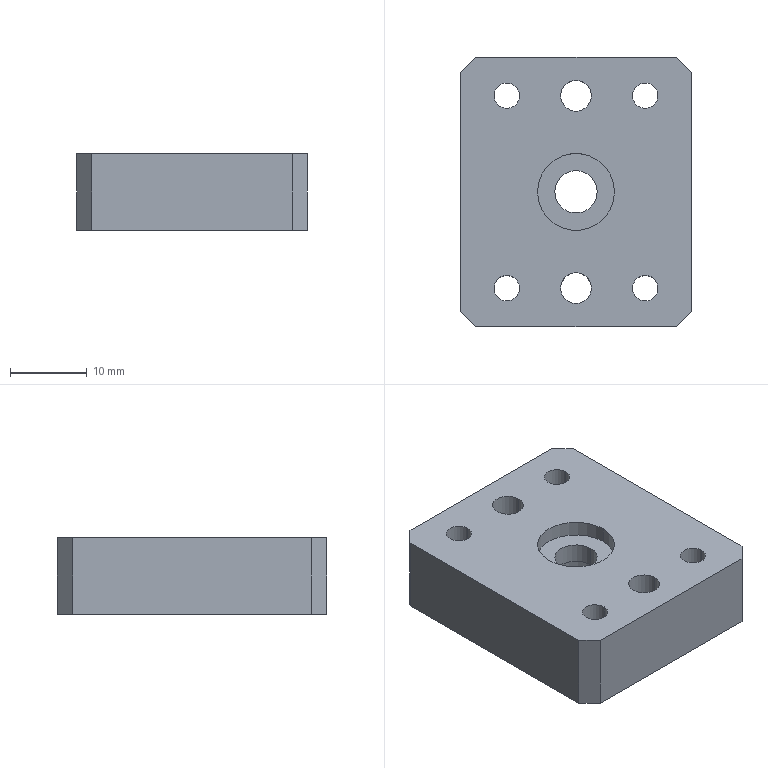Component | SolidWorks | 08-1111-2 | 1 solid | 30 faces | box 30 x 35 x 10 mm | volume 9184 mm3 | cylinder 18 | plane 12 | commonest cylinder face diameters 3.3 x8 4 x4 10 x4 5.5 x2
build123d program:
from build123d import *

# Parameters (mm, degrees)
SKETCH5_W                                       = 35
SKETCH5_H                                       = 30
BOSS_EXTRUDE1_DEPTH                             = 10
SKETCH6_R                                       = 5
CUT_EXTRUDE1_DEPTH                              = 2
M5_HEX_SOCKET_HEAD_CAP_SCREW_CBORE1_D           = 5.5
M5_HEX_SOCKET_HEAD_CAP_SCREW_CBORE1_CBORE_D     = 10
M5_HEX_SOCKET_HEAD_CAP_SCREW_CBORE1_CBORE_DEPTH = 5.4
M4_TAPPED_HOLE1_D                               = 3.3
SIZE_MM_DOWEL_PIN_HOLE_1_D                      = 4
CHAMFER1_SIZE                                   = 2


with BuildPart() as part:
    # Sketch5 → Boss-Extrude1 (new body)
    with BuildSketch(Plane(origin=(0, 0, 0), x_dir=(1, 0, 0), z_dir=(0, 1, 0))):
        Rectangle(SKETCH5_W, SKETCH5_H)
    extrude(amount=BOSS_EXTRUDE1_DEPTH)

    # Sketch6 → Cut-Extrude1 (cut)
    with BuildSketch(Plane.XZ):
        with Locations(Location((0, 0, 0), (0, 0, 270))):
            Circle(SKETCH6_R)
    extrude(amount=-CUT_EXTRUDE1_DEPTH, mode=Mode.SUBTRACT)

    # M5 Hex Socket Head Cap Screw CBORE1 (through all)
    with Locations(Plane(origin=(0, 10, 0), x_dir=(1, 0, 0), z_dir=(0, 1, 0))):
        with Locations((0, 0)):
            CounterBoreHole(M5_HEX_SOCKET_HEAD_CAP_SCREW_CBORE1_D / 2, M5_HEX_SOCKET_HEAD_CAP_SCREW_CBORE1_CBORE_D / 2, M5_HEX_SOCKET_HEAD_CAP_SCREW_CBORE1_CBORE_DEPTH)

    # M4 Tapped Hole1 (through all)
    with Locations(Plane(origin=(0, 10, 0), x_dir=(1, 0, 0), z_dir=(0, 1, 0))):
        with Locations((0, 0), (12.5, 9), (-12.5, -9), (-12.5, 9), (12.5, -9)):
            Hole(M4_TAPPED_HOLE1_D / 2)

    # Size mm Dowel Pin Hole 1 (through all)
    with Locations(Plane(origin=(0, 10, 0), x_dir=(1, 0, 0), z_dir=(0, 1, 0))):
        with Locations((12.5, 0), (-12.5, 0)):
            Hole(SIZE_MM_DOWEL_PIN_HOLE_1_D / 2)

    # Chamfer1
    chamfer1_edges = [part.edges().sort_by_distance(p)[0] for p in [
        (-17.5, 5, -15),
        (17.5, 5, -15),
        (17.5, 5, 15),
        (-17.5, 5, 15),
    ]]
    chamfer(chamfer1_edges, length=CHAMFER1_SIZE)


solid = part.part

# Placed as in the assembly
solid = solid.moved(Location((63.928, 474.724, 1292.056), (-90, 90, 0)))
STEP:
#1=CARTESIAN_POINT('',(2.596,19.182,50.868));
#2=VERTEX_POINT('',#1);
#3=CARTESIAN_POINT('',(2.438,19.182,50.868));
#4=VERTEX_POINT('',#3);
#5=CARTESIAN_POINT('',(2.517,19.182,50.868));
#6=DIRECTION('',(-0.,0.,-1.));
#7=DIRECTION('',(-1.,0.,0.));
#8=AXIS2_PLACEMENT_3D('',#5,#6,#7);
#9=CIRCLE('',#8,0.07874);
#10=EDGE_CURVE('',#2,#4,#9,.T.);
#11=ORIENTED_EDGE('',*,*,#10,.F.);
#12=CARTESIAN_POINT('',(2.596,19.182,50.475));
#13=VERTEX_POINT('',#12);
#14=CARTESIAN_POINT('',(2.596,19.182,50.475));
#15=DIRECTION('',(-0.,0.,-1.));
#16=VECTOR('',#15,39.37);
#17=LINE('',#14,#16);
#18=EDGE_CURVE('',#2,#13,#17,.T.);
#19=ORIENTED_EDGE('',*,*,#18,.T.);
#20=CARTESIAN_POINT('',(2.438,19.182,50.475));
#21=VERTEX_POINT('',#20);
#22=CARTESIAN_POINT('',(2.517,19.182,50.475));
#23=DIRECTION('',(-0.,0.,-1.));
#24=DIRECTION('',(-1.,0.,0.));
#25=AXIS2_PLACEMENT_3D('',#22,#23,#24);
#26=CIRCLE('',#25,0.07874);
#27=EDGE_CURVE('',#13,#21,#26,.T.);
#28=ORIENTED_EDGE('',*,*,#27,.T.);
#29=CARTESIAN_POINT('',(2.438,19.182,50.475));
#30=DIRECTION('',(-0.,0.,-1.));
#31=VECTOR('',#30,39.37);
#32=LINE('',#29,#31);
#33=EDGE_CURVE('',#4,#21,#32,.T.);
#34=ORIENTED_EDGE('',*,*,#33,.F.);
#35=EDGE_LOOP('',(#11,#19,#28,#34));
#36=FACE_OUTER_BOUND('',#35,.T.);
#37=CARTESIAN_POINT('',(2.517,19.182,50.475));
#38=DIRECTION('',(-0.,0.,-1.));
#39=DIRECTION('',(-1.,0.,0.));
#40=AXIS2_PLACEMENT_3D('',#37,#38,#39);
#41=CYLINDRICAL_SURFACE('',#40,0.07874);
#42=ADVANCED_FACE('',(#36),#41,.F.);
#43=CARTESIAN_POINT('',(2.596,18.198,50.868));
#44=VERTEX_POINT('',#43);
#45=CARTESIAN_POINT('',(2.438,18.198,50.868));
#46=VERTEX_POINT('',#45);
#47=CARTESIAN_POINT('',(2.517,18.198,50.868));
#48=DIRECTION('',(-0.,0.,-1.));
#49=DIRECTION('',(-1.,0.,0.));
#50=AXIS2_PLACEMENT_3D('',#47,#48,#49);
#51=CIRCLE('',#50,0.07874);
#52=EDGE_CURVE('',#44,#46,#51,.T.);
#53=ORIENTED_EDGE('',*,*,#52,.F.);
#54=CARTESIAN_POINT('',(2.596,18.198,50.475));
#55=VERTEX_POINT('',#54);
#56=CARTESIAN_POINT('',(2.596,18.198,50.475));
#57=DIRECTION('',(-0.,0.,-1.));
#58=VECTOR('',#57,39.37);
#59=LINE('',#56,#58);
#60=EDGE_CURVE('',#44,#55,#59,.T.);
#61=ORIENTED_EDGE('',*,*,#60,.T.);
#62=CARTESIAN_POINT('',(2.438,18.198,50.475));
#63=VERTEX_POINT('',#62);
#64=CARTESIAN_POINT('',(2.517,18.198,50.475));
#65=DIRECTION('',(-0.,0.,-1.));
#66=DIRECTION('',(-1.,0.,0.));
#67=AXIS2_PLACEMENT_3D('',#64,#65,#66);
#68=CIRCLE('',#67,0.07874);
#69=EDGE_CURVE('',#55,#63,#68,.T.);
#70=ORIENTED_EDGE('',*,*,#69,.T.);
#71=CARTESIAN_POINT('',(2.438,18.198,50.475));
#72=DIRECTION('',(-0.,0.,-1.));
#73=VECTOR('',#72,39.37);
#74=LINE('',#71,#73);
#75=EDGE_CURVE('',#46,#63,#74,.T.);
#76=ORIENTED_EDGE('',*,*,#75,.F.);
#77=EDGE_LOOP('',(#53,#61,#70,#76));
#78=FACE_OUTER_BOUND('',#77,.T.);
#79=CARTESIAN_POINT('',(2.517,18.198,50.475));
#80=DIRECTION('',(-0.,0.,-1.));
#81=DIRECTION('',(-1.,0.,0.));
#82=AXIS2_PLACEMENT_3D('',#79,#80,#81);
#83=CYLINDRICAL_SURFACE('',#82,0.07874);
#84=ADVANCED_FACE('',(#78),#83,.F.);
#85=CARTESIAN_POINT('',(2.936,19.182,50.868));
#86=VERTEX_POINT('',#85);
#87=CARTESIAN_POINT('',(2.806,19.182,50.868));
#88=VERTEX_POINT('',#87);
#89=CARTESIAN_POINT('',(2.871,19.182,50.868));
#90=DIRECTION('',(-0.,0.,-1.));
#91=DIRECTION('',(-1.,0.,0.));
#92=AXIS2_PLACEMENT_3D('',#89,#90,#91);
#93=CIRCLE('',#92,0.06496);
#94=EDGE_CURVE('',#86,#88,#93,.T.);
#95=ORIENTED_EDGE('',*,*,#94,.F.);
#96=CARTESIAN_POINT('',(2.936,19.182,50.475));
#97=VERTEX_POINT('',#96);
#98=CARTESIAN_POINT('',(2.936,19.182,50.475));
#99=DIRECTION('',(-0.,0.,-1.));
#100=VECTOR('',#99,39.37);
#101=LINE('',#98,#100);
#102=EDGE_CURVE('',#86,#97,#101,.T.);
#103=ORIENTED_EDGE('',*,*,#102,.T.);
#104=CARTESIAN_POINT('',(2.806,19.182,50.475));
#105=VERTEX_POINT('',#104);
#106=CARTESIAN_POINT('',(2.871,19.182,50.475));
#107=DIRECTION('',(-0.,0.,-1.));
#108=DIRECTION('',(-1.,0.,0.));
#109=AXIS2_PLACEMENT_3D('',#106,#107,#108);
#110=CIRCLE('',#109,0.06496);
#111=EDGE_CURVE('',#97,#105,#110,.T.);
#112=ORIENTED_EDGE('',*,*,#111,.T.);
#113=CARTESIAN_POINT('',(2.806,19.182,50.475));
#114=DIRECTION('',(-0.,0.,-1.));
#115=VECTOR('',#114,39.37);
#116=LINE('',#113,#115);
#117=EDGE_CURVE('',#88,#105,#116,.T.);
#118=ORIENTED_EDGE('',*,*,#117,.F.);
#119=EDGE_LOOP('',(#95,#103,#112,#118));
#120=FACE_OUTER_BOUND('',#119,.T.);
#121=CARTESIAN_POINT('',(2.871,19.182,50.475));
#122=DIRECTION('',(-0.,0.,-1.));
#123=DIRECTION('',(-1.,0.,0.));
#124=AXIS2_PLACEMENT_3D('',#121,#122,#123);
#125=CYLINDRICAL_SURFACE('',#124,0.06496);
#126=ADVANCED_FACE('',(#120),#125,.F.);
#127=CARTESIAN_POINT('',(2.227,18.198,50.868));
#128=VERTEX_POINT('',#127);
#129=CARTESIAN_POINT('',(2.098,18.198,50.868));
#130=VERTEX_POINT('',#129);
#131=CARTESIAN_POINT('',(2.163,18.198,50.868));
#132=DIRECTION('',(-0.,0.,-1.));
#133=DIRECTION('',(-1.,0.,0.));
#134=AXIS2_PLACEMENT_3D('',#131,#132,#133);
#135=CIRCLE('',#134,0.06496);
#136=EDGE_CURVE('',#128,#130,#135,.T.);
#137=ORIENTED_EDGE('',*,*,#136,.F.);
#138=CARTESIAN_POINT('',(2.227,18.198,50.475));
#139=VERTEX_POINT('',#138);
#140=CARTESIAN_POINT('',(2.227,18.198,50.475));
#141=DIRECTION('',(-0.,0.,-1.));
#142=VECTOR('',#141,39.37);
#143=LINE('',#140,#142);
#144=EDGE_CURVE('',#128,#139,#143,.T.);
#145=ORIENTED_EDGE('',*,*,#144,.T.);
#146=CARTESIAN_POINT('',(2.098,18.198,50.475));
#147=VERTEX_POINT('',#146);
#148=CARTESIAN_POINT('',(2.163,18.198,50.475));
#149=DIRECTION('',(-0.,0.,-1.));
#150=DIRECTION('',(-1.,0.,0.));
#151=AXIS2_PLACEMENT_3D('',#148,#149,#150);
#152=CIRCLE('',#151,0.06496);
#153=EDGE_CURVE('',#139,#147,#152,.T.);
#154=ORIENTED_EDGE('',*,*,#153,.T.);
#155=CARTESIAN_POINT('',(2.098,18.198,50.475));
#156=DIRECTION('',(-0.,0.,-1.));
#157=VECTOR('',#156,39.37);
#158=LINE('',#155,#157);
#159=EDGE_CURVE('',#130,#147,#158,.T.);
#160=ORIENTED_EDGE('',*,*,#159,.F.);
#161=EDGE_LOOP('',(#137,#145,#154,#160));
#162=FACE_OUTER_BOUND('',#161,.T.);
#163=CARTESIAN_POINT('',(2.163,18.198,50.475));
#164=DIRECTION('',(-0.,0.,-1.));
#165=DIRECTION('',(-1.,0.,0.));
#166=AXIS2_PLACEMENT_3D('',#163,#164,#165);
#167=CYLINDRICAL_SURFACE('',#166,0.06496);
#168=ADVANCED_FACE('',(#162),#167,.F.);
#169=CARTESIAN_POINT('',(2.936,18.198,50.868));
#170=VERTEX_POINT('',#169);
#171=CARTESIAN_POINT('',(2.806,18.198,50.868));
#172=VERTEX_POINT('',#171);
#173=CARTESIAN_POINT('',(2.871,18.198,50.868));
#174=DIRECTION('',(-0.,0.,-1.));
#175=DIRECTION('',(-1.,0.,0.));
#176=AXIS2_PLACEMENT_3D('',#173,#174,#175);
#177=CIRCLE('',#176,0.06496);
#178=EDGE_CURVE('',#170,#172,#177,.T.);
#179=ORIENTED_EDGE('',*,*,#178,.F.);
#180=CARTESIAN_POINT('',(2.936,18.198,50.475));
#181=VERTEX_POINT('',#180);
#182=CARTESIAN_POINT('',(2.936,18.198,50.475));
#183=DIRECTION('',(-0.,0.,-1.));
#184=VECTOR('',#183,39.37);
#185=LINE('',#182,#184);
#186=EDGE_CURVE('',#170,#181,#185,.T.);
#187=ORIENTED_EDGE('',*,*,#186,.T.);
#188=CARTESIAN_POINT('',(2.806,18.198,50.475));
#189=VERTEX_POINT('',#188);
#190=CARTESIAN_POINT('',(2.871,18.198,50.475));
#191=DIRECTION('',(-0.,0.,-1.));
#192=DIRECTION('',(-1.,0.,0.));
#193=AXIS2_PLACEMENT_3D('',#190,#191,#192);
#194=CIRCLE('',#193,0.06496);
#195=EDGE_CURVE('',#181,#189,#194,.T.);
#196=ORIENTED_EDGE('',*,*,#195,.T.);
#197=CARTESIAN_POINT('',(2.806,18.198,50.475));
#198=DIRECTION('',(-0.,0.,-1.));
#199=VECTOR('',#198,39.37);
#200=LINE('',#197,#199);
#201=EDGE_CURVE('',#172,#189,#200,.T.);
#202=ORIENTED_EDGE('',*,*,#201,.F.);
#203=EDGE_LOOP('',(#179,#187,#196,#202));
#204=FACE_OUTER_BOUND('',#203,.T.);
#205=CARTESIAN_POINT('',(2.871,18.198,50.475));
#206=DIRECTION('',(-0.,0.,-1.));
#207=DIRECTION('',(-1.,0.,0.));
#208=AXIS2_PLACEMENT_3D('',#205,#206,#207);
#209=CYLINDRICAL_SURFACE('',#208,0.06496);
#210=ADVANCED_FACE('',(#204),#209,.F.);
#211=CARTESIAN_POINT('',(2.227,19.182,50.868));
#212=VERTEX_POINT('',#211);
#213=CARTESIAN_POINT('',(2.098,19.182,50.868));
#214=VERTEX_POINT('',#213);
#215=CARTESIAN_POINT('',(2.163,19.182,50.868));
#216=DIRECTION('',(-0.,0.,-1.));
#217=DIRECTION('',(-1.,0.,0.));
#218=AXIS2_PLACEMENT_3D('',#215,#216,#217);
#219=CIRCLE('',#218,0.06496);
#220=EDGE_CURVE('',#212,#214,#219,.T.);
#221=ORIENTED_EDGE('',*,*,#220,.F.);
#222=CARTESIAN_POINT('',(2.227,19.182,50.475));
#223=VERTEX_POINT('',#222);
#224=CARTESIAN_POINT('',(2.227,19.182,50.475));
#225=DIRECTION('',(-0.,0.,-1.));
#226=VECTOR('',#225,39.37);
#227=LINE('',#224,#226);
#228=EDGE_CURVE('',#212,#223,#227,.T.);
#229=ORIENTED_EDGE('',*,*,#228,.T.);
#230=CARTESIAN_POINT('',(2.098,19.182,50.475));
#231=VERTEX_POINT('',#230);
#232=CARTESIAN_POINT('',(2.163,19.182,50.475));
#233=DIRECTION('',(-0.,0.,-1.));
#234=DIRECTION('',(-1.,0.,0.));
#235=AXIS2_PLACEMENT_3D('',#232,#233,#234);
#236=CIRCLE('',#235,0.06496);
#237=EDGE_CURVE('',#223,#231,#236,.T.);
#238=ORIENTED_EDGE('',*,*,#237,.T.);
#239=CARTESIAN_POINT('',(2.098,19.182,50.475));
#240=DIRECTION('',(-0.,0.,-1.));
#241=VECTOR('',#240,39.37);
#242=LINE('',#239,#241);
#243=EDGE_CURVE('',#214,#231,#242,.T.);
#244=ORIENTED_EDGE('',*,*,#243,.F.);
#245=EDGE_LOOP('',(#221,#229,#238,#244));
#246=FACE_OUTER_BOUND('',#245,.T.);
#247=CARTESIAN_POINT('',(2.163,19.182,50.475));
#248=DIRECTION('',(-0.,0.,-1.));
#249=DIRECTION('',(-1.,0.,0.));
#250=AXIS2_PLACEMENT_3D('',#247,#248,#249);
#251=CYLINDRICAL_SURFACE('',#250,0.06496);
#252=ADVANCED_FACE('',(#246),#251,.F.);
#253=CARTESIAN_POINT('',(2.714,18.69,50.687));
#254=VERTEX_POINT('',#253);
#255=CARTESIAN_POINT('',(2.32,18.69,50.687));
#256=VERTEX_POINT('',#255);
#257=CARTESIAN_POINT('',(2.517,18.69,50.687));
#258=DIRECTION('',(-0.,0.,-1.));
#259=DIRECTION('',(-1.,0.,0.));
#260=AXIS2_PLACEMENT_3D('',#257,#258,#259);
#261=CIRCLE('',#260,0.1969);
#262=EDGE_CURVE('',#254,#256,#261,.T.);
#263=ORIENTED_EDGE('',*,*,#262,.F.);
#264=CARTESIAN_POINT('',(2.714,18.69,50.475));
#265=VERTEX_POINT('',#264);
#266=CARTESIAN_POINT('',(2.714,18.69,50.475));
#267=DIRECTION('',(-0.,0.,-1.));
#268=VECTOR('',#267,39.37);
#269=LINE('',#266,#268);
#270=EDGE_CURVE('',#254,#265,#269,.T.);
#271=ORIENTED_EDGE('',*,*,#270,.T.);
#272=CARTESIAN_POINT('',(2.32,18.69,50.475));
#273=VERTEX_POINT('',#272);
#274=CARTESIAN_POINT('',(2.517,18.69,50.475));
#275=DIRECTION('',(-0.,0.,-1.));
#276=DIRECTION('',(-1.,0.,0.));
#277=AXIS2_PLACEMENT_3D('',#274,#275,#276);
#278=CIRCLE('',#277,0.1969);
#279=EDGE_CURVE('',#265,#273,#278,.T.);
#280=ORIENTED_EDGE('',*,*,#279,.T.);
#281=CARTESIAN_POINT('',(2.32,18.69,50.475));
#282=DIRECTION('',(-0.,0.,-1.));
#283=VECTOR('',#282,39.37);
#284=LINE('',#281,#283);
#285=EDGE_CURVE('',#256,#273,#284,.T.);
#286=ORIENTED_EDGE('',*,*,#285,.F.);
#287=EDGE_LOOP('',(#263,#271,#280,#286));
#288=FACE_OUTER_BOUND('',#287,.T.);
#289=CARTESIAN_POINT('',(2.517,18.69,50.475));
#290=DIRECTION('',(-0.,0.,-1.));
#291=DIRECTION('',(-1.,0.,0.));
#292=AXIS2_PLACEMENT_3D('',#289,#290,#291);
#293=CYLINDRICAL_SURFACE('',#292,0.1969);
#294=ADVANCED_FACE('',(#288),#293,.F.);
#295=CARTESIAN_POINT('',(2.409,18.69,50.79));
#296=VERTEX_POINT('',#295);
#297=CARTESIAN_POINT('',(2.625,18.69,50.79));
#298=VERTEX_POINT('',#297);
#299=CARTESIAN_POINT('',(2.517,18.69,50.79));
#300=DIRECTION('',(0.,-0.,1.));
#301=DIRECTION('',(1.,0.,0.));
#302=AXIS2_PLACEMENT_3D('',#299,#300,#301);
#303=CIRCLE('',#302,0.1083);
#304=EDGE_CURVE('',#296,#298,#303,.T.);
#305=ORIENTED_EDGE('',*,*,#304,.T.);
#306=CARTESIAN_POINT('',(2.625,18.69,50.687));
#307=VERTEX_POINT('',#306);
#308=CARTESIAN_POINT('',(2.625,18.69,50.475));
#309=DIRECTION('',(-0.,0.,-1.));
#310=VECTOR('',#309,39.37);
#311=LINE('',#308,#310);
#312=EDGE_CURVE('',#298,#307,#311,.T.);
#313=ORIENTED_EDGE('',*,*,#312,.T.);
#314=CARTESIAN_POINT('',(2.409,18.69,50.687));
#315=VERTEX_POINT('',#314);
#316=CARTESIAN_POINT('',(2.517,18.69,50.687));
#317=DIRECTION('',(-0.,0.,-1.));
#318=DIRECTION('',(-1.,0.,0.));
#319=AXIS2_PLACEMENT_3D('',#316,#317,#318);
#320=CIRCLE('',#319,0.1083);
#321=EDGE_CURVE('',#307,#315,#320,.T.);
#322=ORIENTED_EDGE('',*,*,#321,.T.);
#323=CARTESIAN_POINT('',(2.409,18.69,50.475));
#324=DIRECTION('',(-0.,0.,-1.));
#325=VECTOR('',#324,39.37);
#326=LINE('',#323,#325);
#327=EDGE_CURVE('',#296,#315,#326,.T.);
#328=ORIENTED_EDGE('',*,*,#327,.F.);
#329=EDGE_LOOP('',(#305,#313,#322,#328));
#330=FACE_OUTER_BOUND('',#329,.T.);
#331=CARTESIAN_POINT('',(2.517,18.69,50.475));
#332=DIRECTION('',(-0.,0.,-1.));
#333=DIRECTION('',(-1.,0.,0.));
#334=AXIS2_PLACEMENT_3D('',#331,#332,#333);
#335=CYLINDRICAL_SURFACE('',#334,0.1083);
#336=ADVANCED_FACE('',(#330),#335,.F.);
#337=CARTESIAN_POINT('',(2.32,18.69,50.79));
#338=VERTEX_POINT('',#337);
#339=CARTESIAN_POINT('',(2.714,18.69,50.79));
#340=VERTEX_POINT('',#339);
#341=CARTESIAN_POINT('',(2.517,18.69,50.79));
#342=DIRECTION('',(0.,-0.,1.));
#343=DIRECTION('',(1.,0.,0.));
#344=AXIS2_PLACEMENT_3D('',#341,#342,#343);
#345=CIRCLE('',#344,0.1969);
#346=EDGE_CURVE('',#338,#340,#345,.T.);
#347=ORIENTED_EDGE('',*,*,#346,.F.);
#348=CARTESIAN_POINT('',(2.32,18.69,50.868));
#349=VERTEX_POINT('',#348);
#350=CARTESIAN_POINT('',(2.32,18.69,50.79));
#351=DIRECTION('',(0.,-0.,1.));
#352=VECTOR('',#351,39.37);
#353=LINE('',#350,#352);
#354=EDGE_CURVE('',#338,#349,#353,.T.);
#355=ORIENTED_EDGE('',*,*,#354,.T.);
#356=CARTESIAN_POINT('',(2.714,18.69,50.868));
#357=VERTEX_POINT('',#356);
#358=CARTESIAN_POINT('',(2.517,18.69,50.868));
#359=DIRECTION('',(0.,-0.,1.));
#360=DIRECTION('',(1.,0.,0.));
#361=AXIS2_PLACEMENT_3D('',#358,#359,#360);
#362=CIRCLE('',#361,0.1969);
#363=EDGE_CURVE('',#349,#357,#362,.T.);
#364=ORIENTED_EDGE('',*,*,#363,.T.);
#365=CARTESIAN_POINT('',(2.714,18.69,50.79));
#366=DIRECTION('',(0.,-0.,1.));
#367=VECTOR('',#366,39.37);
#368=LINE('',#365,#367);
#369=EDGE_CURVE('',#340,#357,#368,.T.);
#370=ORIENTED_EDGE('',*,*,#369,.F.);
#371=EDGE_LOOP('',(#347,#355,#364,#370));
#372=FACE_OUTER_BOUND('',#371,.T.);
#373=CARTESIAN_POINT('',(2.517,18.69,50.79));
#374=DIRECTION('',(0.,-0.,1.));
#375=DIRECTION('',(1.,0.,0.));
#376=AXIS2_PLACEMENT_3D('',#373,#374,#375);
#377=CYLINDRICAL_SURFACE('',#376,0.1969);
#378=ADVANCED_FACE('',(#372),#377,.F.);
#379=CARTESIAN_POINT('',(3.029,18.001,50.475));
#380=VERTEX_POINT('',#379);
#381=CARTESIAN_POINT('',(2.005,18.001,50.475));
#382=VERTEX_POINT('',#381);
#383=CARTESIAN_POINT('',(1.926,18.001,50.475));
#384=DIRECTION('',(-1.,0.,0.));
#385=VECTOR('',#384,39.37);
#386=LINE('',#383,#385);
#387=EDGE_CURVE('',#380,#382,#386,.T.);
#388=ORIENTED_EDGE('',*,*,#387,.F.);
#389=CARTESIAN_POINT('',(3.029,18.001,50.868));
#390=VERTEX_POINT('',#389);
#391=CARTESIAN_POINT('',(3.029,18.001,50.475));
#392=DIRECTION('',(0.,-0.,1.));
#393=VECTOR('',#392,39.37);
#394=LINE('',#391,#393);
#395=EDGE_CURVE('',#380,#390,#394,.T.);
#396=ORIENTED_EDGE('',*,*,#395,.T.);
#397=CARTESIAN_POINT('',(2.005,18.001,50.868));
#398=VERTEX_POINT('',#397);
#399=CARTESIAN_POINT('',(1.926,18.001,50.868));
#400=DIRECTION('',(-1.,0.,0.));
#401=VECTOR('',#400,39.37);
#402=LINE('',#399,#401);
#403=EDGE_CURVE('',#390,#398,#402,.T.);
#404=ORIENTED_EDGE('',*,*,#403,.T.);
#405=CARTESIAN_POINT('',(2.005,18.001,50.475));
#406=DIRECTION('',(-0.,0.,-1.));
#407=VECTOR('',#406,39.37);
#408=LINE('',#405,#407);
#409=EDGE_CURVE('',#398,#382,#408,.T.);
#410=ORIENTED_EDGE('',*,*,#409,.T.);
#411=EDGE_LOOP('',(#388,#396,#404,#410));
#412=FACE_OUTER_BOUND('',#411,.T.);
#413=CARTESIAN_POINT('',(1.926,18.001,50.475));
#414=DIRECTION('',(0.,1.,0.));
#415=DIRECTION('',(1.,-0.,-0.));
#416=AXIS2_PLACEMENT_3D('',#413,#414,#415);
#417=PLANE('',#416);
#418=ADVANCED_FACE('',(#412),#417,.F.);
#419=CARTESIAN_POINT('',(1.926,18.08,50.868));
#420=VERTEX_POINT('',#419);
#421=CARTESIAN_POINT('',(1.926,19.3,50.868));
#422=VERTEX_POINT('',#421);
#423=CARTESIAN_POINT('',(1.926,19.379,50.868));
#424=DIRECTION('',(-0.,1.,0.));
#425=VECTOR('',#424,39.37);
#426=LINE('',#423,#425);
#427=EDGE_CURVE('',#420,#422,#426,.T.);
#428=ORIENTED_EDGE('',*,*,#427,.T.);
#429=CARTESIAN_POINT('',(1.926,19.3,50.475));
#430=VERTEX_POINT('',#429);
#431=CARTESIAN_POINT('',(1.926,19.3,50.475));
#432=DIRECTION('',(-0.,0.,-1.));
#433=VECTOR('',#432,39.37);
#434=LINE('',#431,#433);
#435=EDGE_CURVE('',#422,#430,#434,.T.);
#436=ORIENTED_EDGE('',*,*,#435,.T.);
#437=CARTESIAN_POINT('',(1.926,18.08,50.475));
#438=VERTEX_POINT('',#437);
#439=CARTESIAN_POINT('',(1.926,19.379,50.475));
#440=DIRECTION('',(-0.,1.,0.));
#441=VECTOR('',#440,39.37);
#442=LINE('',#439,#441);
#443=EDGE_CURVE('',#438,#430,#442,.T.);
#444=ORIENTED_EDGE('',*,*,#443,.F.);
#445=CARTESIAN_POINT('',(1.926,18.08,50.475));
#446=DIRECTION('',(0.,-0.,1.));
#447=VECTOR('',#446,39.37);
#448=LINE('',#445,#447);
#449=EDGE_CURVE('',#438,#420,#448,.T.);
#450=ORIENTED_EDGE('',*,*,#449,.T.);
#451=EDGE_LOOP('',(#428,#436,#444,#450));
#452=FACE_OUTER_BOUND('',#451,.T.);
#453=CARTESIAN_POINT('',(1.926,19.379,50.475));
#454=DIRECTION('',(1.,0.,-0.));
#455=DIRECTION('',(0.,-1.,-0.));
#456=AXIS2_PLACEMENT_3D('',#453,#454,#455);
#457=PLANE('',#456);
#458=ADVANCED_FACE('',(#452),#457,.F.);
#459=CARTESIAN_POINT('',(2.005,19.379,50.868));
#460=VERTEX_POINT('',#459);
#461=CARTESIAN_POINT('',(3.029,19.379,50.868));
#462=VERTEX_POINT('',#461);
#463=CARTESIAN_POINT('',(1.926,19.379,50.868));
#464=DIRECTION('',(1.,-0.,-0.));
#465=VECTOR('',#464,39.37);
#466=LINE('',#463,#465);
#467=EDGE_CURVE('',#460,#462,#466,.T.);
#468=ORIENTED_EDGE('',*,*,#467,.T.);
#469=CARTESIAN_POINT('',(3.029,19.379,50.475));
#470=VERTEX_POINT('',#469);
#471=CARTESIAN_POINT('',(3.029,19.379,50.475));
#472=DIRECTION('',(-0.,0.,-1.));
#473=VECTOR('',#472,39.37);
#474=LINE('',#471,#473);
#475=EDGE_CURVE('',#462,#470,#474,.T.);
#476=ORIENTED_EDGE('',*,*,#475,.T.);
#477=CARTESIAN_POINT('',(2.005,19.379,50.475));
#478=VERTEX_POINT('',#477);
#479=CARTESIAN_POINT('',(1.926,19.379,50.475));
#480=DIRECTION('',(1.,-0.,-0.));
#481=VECTOR('',#480,39.37);
#482=LINE('',#479,#481);
#483=EDGE_CURVE('',#478,#470,#482,.T.);
#484=ORIENTED_EDGE('',*,*,#483,.F.);
#485=CARTESIAN_POINT('',(2.005,19.379,50.475));
#486=DIRECTION('',(0.,-0.,1.));
#487=VECTOR('',#486,39.37);
#488=LINE('',#485,#487);
#489=EDGE_CURVE('',#478,#460,#488,.T.);
#490=ORIENTED_EDGE('',*,*,#489,.T.);
#491=EDGE_LOOP('',(#468,#476,#484,#490));
#492=FACE_OUTER_BOUND('',#491,.T.);
#493=CARTESIAN_POINT('',(1.926,19.379,50.475));
#494=DIRECTION('',(-0.,-1.,-0.));
#495=DIRECTION('',(-1.,0.,0.));
#496=AXIS2_PLACEMENT_3D('',#493,#494,#495);
#497=PLANE('',#496);
#498=ADVANCED_FACE('',(#492),#497,.F.);
#499=CARTESIAN_POINT('',(3.107,19.3,50.868));
#500=VERTEX_POINT('',#499);
#501=CARTESIAN_POINT('',(3.107,18.08,50.868));
#502=VERTEX_POINT('',#501);
#503=CARTESIAN_POINT('',(3.107,19.379,50.868));
#504=DIRECTION('',(0.,-1.,-0.));
#505=VECTOR('',#504,39.37);
#506=LINE('',#503,#505);
#507=EDGE_CURVE('',#500,#502,#506,.T.);
#508=ORIENTED_EDGE('',*,*,#507,.T.);
#509=CARTESIAN_POINT('',(3.107,18.08,50.475));
#510=VERTEX_POINT('',#509);
#511=CARTESIAN_POINT('',(3.107,18.08,50.475));
#512=DIRECTION('',(-0.,0.,-1.));
#513=VECTOR('',#512,39.37);
#514=LINE('',#511,#513);
#515=EDGE_CURVE('',#502,#510,#514,.T.);
#516=ORIENTED_EDGE('',*,*,#515,.T.);
#517=CARTESIAN_POINT('',(3.107,19.3,50.475));
#518=VERTEX_POINT('',#517);
#519=CARTESIAN_POINT('',(3.107,19.379,50.475));
#520=DIRECTION('',(0.,-1.,-0.));
#521=VECTOR('',#520,39.37);
#522=LINE('',#519,#521);
#523=EDGE_CURVE('',#518,#510,#522,.T.);
#524=ORIENTED_EDGE('',*,*,#523,.F.);
#525=CARTESIAN_POINT('',(3.107,19.3,50.475));
#526=DIRECTION('',(0.,-0.,1.));
#527=VECTOR('',#526,39.37);
#528=LINE('',#525,#527);
#529=EDGE_CURVE('',#518,#500,#528,.T.);
#530=ORIENTED_EDGE('',*,*,#529,.T.);
#531=EDGE_LOOP('',(#508,#516,#524,#530));
#532=FACE_OUTER_BOUND('',#531,.T.);
#533=CARTESIAN_POINT('',(3.107,19.379,50.475));
#534=DIRECTION('',(-1.,-0.,0.));
#535=DIRECTION('',(-0.,1.,0.));
#536=AXIS2_PLACEMENT_3D('',#533,#534,#535);
#537=PLANE('',#536);
#538=ADVANCED_FACE('',(#532),#537,.F.);
#539=CARTESIAN_POINT('',(2.517,19.182,50.475));
#540=DIRECTION('',(-0.,0.,-1.));
#541=DIRECTION('',(-1.,0.,0.));
#542=AXIS2_PLACEMENT_3D('',#539,#540,#541);
#543=CIRCLE('',#542,0.07874);
#544=EDGE_CURVE('',#21,#13,#543,.T.);
#545=ORIENTED_EDGE('',*,*,#544,.F.);
#546=ORIENTED_EDGE('',*,*,#27,.F.);
#547=EDGE_LOOP('',(#545,#546));
#548=FACE_BOUND('',#547,.T.);
#549=CARTESIAN_POINT('',(2.517,18.198,50.475));
#550=DIRECTION('',(-0.,0.,-1.));
#551=DIRECTION('',(-1.,0.,0.));
#552=AXIS2_PLACEMENT_3D('',#549,#550,#551);
#553=CIRCLE('',#552,0.07874);
#554=EDGE_CURVE('',#63,#55,#553,.T.);
#555=ORIENTED_EDGE('',*,*,#554,.F.);
#556=ORIENTED_EDGE('',*,*,#69,.F.);
#557=EDGE_LOOP('',(#555,#556));
#558=FACE_BOUND('',#557,.T.);
#559=CARTESIAN_POINT('',(2.871,19.182,50.475));
#560=DIRECTION('',(-0.,0.,-1.));
#561=DIRECTION('',(-1.,0.,0.));
#562=AXIS2_PLACEMENT_3D('',#559,#560,#561);
#563=CIRCLE('',#562,0.06496);
#564=EDGE_CURVE('',#105,#97,#563,.T.);
#565=ORIENTED_EDGE('',*,*,#564,.F.);
#566=ORIENTED_EDGE('',*,*,#111,.F.);
#567=EDGE_LOOP('',(#565,#566));
#568=FACE_BOUND('',#567,.T.);
#569=CARTESIAN_POINT('',(2.163,18.198,50.475));
#570=DIRECTION('',(-0.,0.,-1.));
#571=DIRECTION('',(-1.,0.,0.));
#572=AXIS2_PLACEMENT_3D('',#569,#570,#571);
#573=CIRCLE('',#572,0.06496);
#574=EDGE_CURVE('',#147,#139,#573,.T.);
#575=ORIENTED_EDGE('',*,*,#574,.F.);
#576=ORIENTED_EDGE('',*,*,#153,.F.);
#577=EDGE_LOOP('',(#575,#576));
#578=FACE_BOUND('',#577,.T.);
#579=CARTESIAN_POINT('',(2.871,18.198,50.475));
#580=DIRECTION('',(-0.,0.,-1.));
#581=DIRECTION('',(-1.,0.,0.));
#582=AXIS2_PLACEMENT_3D('',#579,#580,#581);
#583=CIRCLE('',#582,0.06496);
#584=EDGE_CURVE('',#189,#181,#583,.T.);
#585=ORIENTED_EDGE('',*,*,#584,.F.);
#586=ORIENTED_EDGE('',*,*,#195,.F.);
#587=EDGE_LOOP('',(#585,#586));
#588=FACE_BOUND('',#587,.T.);
#589=CARTESIAN_POINT('',(2.163,19.182,50.475));
#590=DIRECTION('',(-0.,0.,-1.));
#591=DIRECTION('',(-1.,0.,0.));
#592=AXIS2_PLACEMENT_3D('',#589,#590,#591);
#593=CIRCLE('',#592,0.06496);
#594=EDGE_CURVE('',#231,#223,#593,.T.);
#595=ORIENTED_EDGE('',*,*,#594,.F.);
#596=ORIENTED_EDGE('',*,*,#237,.F.);
#597=EDGE_LOOP('',(#595,#596));
#598=FACE_BOUND('',#597,.T.);
#599=CARTESIAN_POINT('',(2.517,18.69,50.475));
#600=DIRECTION('',(-0.,0.,-1.));
#601=DIRECTION('',(-1.,0.,0.));
#602=AXIS2_PLACEMENT_3D('',#599,#600,#601);
#603=CIRCLE('',#602,0.1969);
#604=EDGE_CURVE('',#273,#265,#603,.T.);
#605=ORIENTED_EDGE('',*,*,#604,.F.);
#606=ORIENTED_EDGE('',*,*,#279,.F.);
#607=EDGE_LOOP('',(#605,#606));
#608=FACE_BOUND('',#607,.T.);
#609=ORIENTED_EDGE('',*,*,#523,.T.);
#610=CARTESIAN_POINT('',(3.117,18.09,50.475));
#611=DIRECTION('',(-0.7071,-0.7071,0.));
#612=VECTOR('',#611,39.37);
#613=LINE('',#610,#612);
#614=EDGE_CURVE('',#510,#380,#613,.T.);
#615=ORIENTED_EDGE('',*,*,#614,.T.);
#616=ORIENTED_EDGE('',*,*,#387,.T.);
#617=CARTESIAN_POINT('',(1.916,18.09,50.475));
#618=DIRECTION('',(-0.7071,0.7071,0.));
#619=VECTOR('',#618,39.37);
#620=LINE('',#617,#619);
#621=EDGE_CURVE('',#382,#438,#620,.T.);
#622=ORIENTED_EDGE('',*,*,#621,.T.);
#623=ORIENTED_EDGE('',*,*,#443,.T.);
#624=CARTESIAN_POINT('',(1.916,19.29,50.475));
#625=DIRECTION('',(0.7071,0.7071,-0.));
#626=VECTOR('',#625,39.37);
#627=LINE('',#624,#626);
#628=EDGE_CURVE('',#430,#478,#627,.T.);
#629=ORIENTED_EDGE('',*,*,#628,.T.);
#630=ORIENTED_EDGE('',*,*,#483,.T.);
#631=CARTESIAN_POINT('',(3.117,19.29,50.475));
#632=DIRECTION('',(0.7071,-0.7071,-0.));
#633=VECTOR('',#632,39.37);
#634=LINE('',#631,#633);
#635=EDGE_CURVE('',#470,#518,#634,.T.);
#636=ORIENTED_EDGE('',*,*,#635,.T.);
#637=EDGE_LOOP('',(#609,#615,#616,#622,#623,#629,#630,#636));
#638=FACE_OUTER_BOUND('',#637,.T.);
#639=CARTESIAN_POINT('',(2.517,18.69,50.475));
#640=DIRECTION('',(-0.,0.,-1.));
#641=DIRECTION('',(-1.,0.,0.));
#642=AXIS2_PLACEMENT_3D('',#639,#640,#641);
#643=PLANE('',#642);
#644=ADVANCED_FACE('',(#548,#558,#568,#578,#588,#598,#608,#638),#643,.T.);
#645=CARTESIAN_POINT('',(2.517,19.182,50.868));
#646=DIRECTION('',(-0.,0.,-1.));
#647=DIRECTION('',(-1.,0.,0.));
#648=AXIS2_PLACEMENT_3D('',#645,#646,#647);
#649=CIRCLE('',#648,0.07874);
#650=EDGE_CURVE('',#4,#2,#649,.T.);
#651=ORIENTED_EDGE('',*,*,#650,.T.);
#652=ORIENTED_EDGE('',*,*,#10,.T.);
#653=EDGE_LOOP('',(#651,#652));
#654=FACE_BOUND('',#653,.T.);
#655=CARTESIAN_POINT('',(2.517,18.198,50.868));
#656=DIRECTION('',(-0.,0.,-1.));
#657=DIRECTION('',(-1.,0.,0.));
#658=AXIS2_PLACEMENT_3D('',#655,#656,#657);
#659=CIRCLE('',#658,0.07874);
#660=EDGE_CURVE('',#46,#44,#659,.T.);
#661=ORIENTED_EDGE('',*,*,#660,.T.);
#662=ORIENTED_EDGE('',*,*,#52,.T.);
#663=EDGE_LOOP('',(#661,#662));
#664=FACE_BOUND('',#663,.T.);
#665=CARTESIAN_POINT('',(2.871,19.182,50.868));
#666=DIRECTION('',(-0.,0.,-1.));
#667=DIRECTION('',(-1.,0.,0.));
#668=AXIS2_PLACEMENT_3D('',#665,#666,#667);
#669=CIRCLE('',#668,0.06496);
#670=EDGE_CURVE('',#88,#86,#669,.T.);
#671=ORIENTED_EDGE('',*,*,#670,.T.);
#672=ORIENTED_EDGE('',*,*,#94,.T.);
#673=EDGE_LOOP('',(#671,#672));
#674=FACE_BOUND('',#673,.T.);
#675=CARTESIAN_POINT('',(2.163,18.198,50.868));
#676=DIRECTION('',(-0.,0.,-1.));
#677=DIRECTION('',(-1.,0.,0.));
#678=AXIS2_PLACEMENT_3D('',#675,#676,#677);
#679=CIRCLE('',#678,0.06496);
#680=EDGE_CURVE('',#130,#128,#679,.T.);
#681=ORIENTED_EDGE('',*,*,#680,.T.);
#682=ORIENTED_EDGE('',*,*,#136,.T.);
#683=EDGE_LOOP('',(#681,#682));
#684=FACE_BOUND('',#683,.T.);
#685=CARTESIAN_POINT('',(2.871,18.198,50.868));
#686=DIRECTION('',(-0.,0.,-1.));
#687=DIRECTION('',(-1.,0.,0.));
#688=AXIS2_PLACEMENT_3D('',#685,#686,#687);
#689=CIRCLE('',#688,0.06496);
#690=EDGE_CURVE('',#172,#170,#689,.T.);
#691=ORIENTED_EDGE('',*,*,#690,.T.);
#692=ORIENTED_EDGE('',*,*,#178,.T.);
#693=EDGE_LOOP('',(#691,#692));
#694=FACE_BOUND('',#693,.T.);
#695=CARTESIAN_POINT('',(2.163,19.182,50.868));
#696=DIRECTION('',(-0.,0.,-1.));
#697=DIRECTION('',(-1.,0.,0.));
#698=AXIS2_PLACEMENT_3D('',#695,#696,#697);
#699=CIRCLE('',#698,0.06496);
#700=EDGE_CURVE('',#214,#212,#699,.T.);
#701=ORIENTED_EDGE('',*,*,#700,.T.);
#702=ORIENTED_EDGE('',*,*,#220,.T.);
#703=EDGE_LOOP('',(#701,#702));
#704=FACE_BOUND('',#703,.T.);
#705=CARTESIAN_POINT('',(2.517,18.69,50.868));
#706=DIRECTION('',(0.,-0.,1.));
#707=DIRECTION('',(1.,0.,0.));
#708=AXIS2_PLACEMENT_3D('',#705,#706,#707);
#709=CIRCLE('',#708,0.1969);
#710=EDGE_CURVE('',#357,#349,#709,.T.);
#711=ORIENTED_EDGE('',*,*,#710,.F.);
#712=ORIENTED_EDGE('',*,*,#363,.F.);
#713=EDGE_LOOP('',(#711,#712));
#714=FACE_BOUND('',#713,.T.);
#715=ORIENTED_EDGE('',*,*,#403,.F.);
#716=CARTESIAN_POINT('',(3.029,18.001,50.868));
#717=DIRECTION('',(0.7071,0.7071,-0.));
#718=VECTOR('',#717,39.37);
#719=LINE('',#716,#718);
#720=EDGE_CURVE('',#390,#502,#719,.T.);
#721=ORIENTED_EDGE('',*,*,#720,.T.);
#722=ORIENTED_EDGE('',*,*,#507,.F.);
#723=CARTESIAN_POINT('',(3.107,19.3,50.868));
#724=DIRECTION('',(-0.7071,0.7071,0.));
#725=VECTOR('',#724,39.37);
#726=LINE('',#723,#725);
#727=EDGE_CURVE('',#500,#462,#726,.T.);
#728=ORIENTED_EDGE('',*,*,#727,.T.);
#729=ORIENTED_EDGE('',*,*,#467,.F.);
#730=CARTESIAN_POINT('',(2.005,19.379,50.868));
#731=DIRECTION('',(-0.7071,-0.7071,0.));
#732=VECTOR('',#731,39.37);
#733=LINE('',#730,#732);
#734=EDGE_CURVE('',#460,#422,#733,.T.);
#735=ORIENTED_EDGE('',*,*,#734,.T.);
#736=ORIENTED_EDGE('',*,*,#427,.F.);
#737=CARTESIAN_POINT('',(1.926,18.08,50.868));
#738=DIRECTION('',(0.7071,-0.7071,-0.));
#739=VECTOR('',#738,39.37);
#740=LINE('',#737,#739);
#741=EDGE_CURVE('',#420,#398,#740,.T.);
#742=ORIENTED_EDGE('',*,*,#741,.T.);
#743=EDGE_LOOP('',(#715,#721,#722,#728,#729,#735,#736,#742));
#744=FACE_OUTER_BOUND('',#743,.T.);
#745=CARTESIAN_POINT('',(2.517,18.69,50.868));
#746=DIRECTION('',(-0.,0.,-1.));
#747=DIRECTION('',(-1.,0.,0.));
#748=AXIS2_PLACEMENT_3D('',#745,#746,#747);
#749=PLANE('',#748);
#750=ADVANCED_FACE('',(#654,#664,#674,#684,#694,#704,#714,#744),#749,.F.);
#751=ORIENTED_EDGE('',*,*,#354,.F.);
#752=CARTESIAN_POINT('',(2.517,18.69,50.79));
#753=DIRECTION('',(0.,-0.,1.));
#754=DIRECTION('',(1.,0.,0.));
#755=AXIS2_PLACEMENT_3D('',#752,#753,#754);
#756=CIRCLE('',#755,0.1969);
#757=EDGE_CURVE('',#340,#338,#756,.T.);
#758=ORIENTED_EDGE('',*,*,#757,.F.);
#759=ORIENTED_EDGE('',*,*,#369,.T.);
#760=ORIENTED_EDGE('',*,*,#710,.T.);
#761=EDGE_LOOP('',(#751,#758,#759,#760));
#762=FACE_OUTER_BOUND('',#761,.T.);
#763=CARTESIAN_POINT('',(2.517,18.69,50.79));
#764=DIRECTION('',(0.,-0.,1.));
#765=DIRECTION('',(1.,0.,0.));
#766=AXIS2_PLACEMENT_3D('',#763,#764,#765);
#767=CYLINDRICAL_SURFACE('',#766,0.1969);
#768=ADVANCED_FACE('',(#762),#767,.F.);
#769=ORIENTED_EDGE('',*,*,#304,.F.);
#770=CARTESIAN_POINT('',(2.517,18.69,50.79));
#771=DIRECTION('',(0.,-0.,1.));
#772=DIRECTION('',(1.,0.,0.));
#773=AXIS2_PLACEMENT_3D('',#770,#771,#772);
#774=CIRCLE('',#773,0.1083);
#775=EDGE_CURVE('',#298,#296,#774,.T.);
#776=ORIENTED_EDGE('',*,*,#775,.F.);
#777=EDGE_LOOP('',(#769,#776));
#778=FACE_BOUND('',#777,.T.);
#779=ORIENTED_EDGE('',*,*,#757,.T.);
#780=ORIENTED_EDGE('',*,*,#346,.T.);
#781=EDGE_LOOP('',(#779,#780));
#782=FACE_OUTER_BOUND('',#781,.T.);
#783=CARTESIAN_POINT('',(2.517,18.69,50.79));
#784=DIRECTION('',(0.,-0.,1.));
#785=DIRECTION('',(1.,-0.,-0.));
#786=AXIS2_PLACEMENT_3D('',#783,#784,#785);
#787=PLANE('',#786);
#788=ADVANCED_FACE('',(#778,#782),#787,.T.);
#789=ORIENTED_EDGE('',*,*,#312,.F.);
#790=ORIENTED_EDGE('',*,*,#775,.T.);
#791=ORIENTED_EDGE('',*,*,#327,.T.);
#792=CARTESIAN_POINT('',(2.517,18.69,50.687));
#793=DIRECTION('',(-0.,0.,-1.));
#794=DIRECTION('',(-1.,0.,0.));
#795=AXIS2_PLACEMENT_3D('',#792,#793,#794);
#796=CIRCLE('',#795,0.1083);
#797=EDGE_CURVE('',#315,#307,#796,.T.);
#798=ORIENTED_EDGE('',*,*,#797,.T.);
#799=EDGE_LOOP('',(#789,#790,#791,#798));
#800=FACE_OUTER_BOUND('',#799,.T.);
#801=CARTESIAN_POINT('',(2.517,18.69,50.475));
#802=DIRECTION('',(-0.,0.,-1.));
#803=DIRECTION('',(-1.,0.,0.));
#804=AXIS2_PLACEMENT_3D('',#801,#802,#803);
#805=CYLINDRICAL_SURFACE('',#804,0.1083);
#806=ADVANCED_FACE('',(#800),#805,.F.);
#807=ORIENTED_EDGE('',*,*,#797,.F.);
#808=ORIENTED_EDGE('',*,*,#321,.F.);
#809=EDGE_LOOP('',(#807,#808));
#810=FACE_BOUND('',#809,.T.);
#811=CARTESIAN_POINT('',(2.517,18.69,50.687));
#812=DIRECTION('',(-0.,0.,-1.));
#813=DIRECTION('',(-1.,0.,0.));
#814=AXIS2_PLACEMENT_3D('',#811,#812,#813);
#815=CIRCLE('',#814,0.1969);
#816=EDGE_CURVE('',#256,#254,#815,.T.);
#817=ORIENTED_EDGE('',*,*,#816,.T.);
#818=ORIENTED_EDGE('',*,*,#262,.T.);
#819=EDGE_LOOP('',(#817,#818));
#820=FACE_OUTER_BOUND('',#819,.T.);
#821=CARTESIAN_POINT('',(2.517,18.798,50.687));
#822=DIRECTION('',(0.,-0.,1.));
#823=DIRECTION('',(1.,-0.,-0.));
#824=AXIS2_PLACEMENT_3D('',#821,#822,#823);
#825=PLANE('',#824);
#826=ADVANCED_FACE('',(#810,#820),#825,.F.);
#827=ORIENTED_EDGE('',*,*,#270,.F.);
#828=ORIENTED_EDGE('',*,*,#816,.F.);
#829=ORIENTED_EDGE('',*,*,#285,.T.);
#830=ORIENTED_EDGE('',*,*,#604,.T.);
#831=EDGE_LOOP('',(#827,#828,#829,#830));
#832=FACE_OUTER_BOUND('',#831,.T.);
#833=CARTESIAN_POINT('',(2.517,18.69,50.475));
#834=DIRECTION('',(-0.,0.,-1.));
#835=DIRECTION('',(-1.,0.,0.));
#836=AXIS2_PLACEMENT_3D('',#833,#834,#835);
#837=CYLINDRICAL_SURFACE('',#836,0.1969);
#838=ADVANCED_FACE('',(#832),#837,.F.);
#839=ORIENTED_EDGE('',*,*,#228,.F.);
#840=ORIENTED_EDGE('',*,*,#700,.F.);
#841=ORIENTED_EDGE('',*,*,#243,.T.);
#842=ORIENTED_EDGE('',*,*,#594,.T.);
#843=EDGE_LOOP('',(#839,#840,#841,#842));
#844=FACE_OUTER_BOUND('',#843,.T.);
#845=CARTESIAN_POINT('',(2.163,19.182,50.475));
#846=DIRECTION('',(-0.,0.,-1.));
#847=DIRECTION('',(-1.,0.,0.));
#848=AXIS2_PLACEMENT_3D('',#845,#846,#847);
#849=CYLINDRICAL_SURFACE('',#848,0.06496);
#850=ADVANCED_FACE('',(#844),#849,.F.);
#851=ORIENTED_EDGE('',*,*,#186,.F.);
#852=ORIENTED_EDGE('',*,*,#690,.F.);
#853=ORIENTED_EDGE('',*,*,#201,.T.);
#854=ORIENTED_EDGE('',*,*,#584,.T.);
#855=EDGE_LOOP('',(#851,#852,#853,#854));
#856=FACE_OUTER_BOUND('',#855,.T.);
#857=CARTESIAN_POINT('',(2.871,18.198,50.475));
#858=DIRECTION('',(-0.,0.,-1.));
#859=DIRECTION('',(-1.,0.,0.));
#860=AXIS2_PLACEMENT_3D('',#857,#858,#859);
#861=CYLINDRICAL_SURFACE('',#860,0.06496);
#862=ADVANCED_FACE('',(#856),#861,.F.);
#863=ORIENTED_EDGE('',*,*,#144,.F.);
#864=ORIENTED_EDGE('',*,*,#680,.F.);
#865=ORIENTED_EDGE('',*,*,#159,.T.);
#866=ORIENTED_EDGE('',*,*,#574,.T.);
#867=EDGE_LOOP('',(#863,#864,#865,#866));
#868=FACE_OUTER_BOUND('',#867,.T.);
#869=CARTESIAN_POINT('',(2.163,18.198,50.475));
#870=DIRECTION('',(-0.,0.,-1.));
#871=DIRECTION('',(-1.,0.,0.));
#872=AXIS2_PLACEMENT_3D('',#869,#870,#871);
#873=CYLINDRICAL_SURFACE('',#872,0.06496);
#874=ADVANCED_FACE('',(#868),#873,.F.);
#875=ORIENTED_EDGE('',*,*,#102,.F.);
#876=ORIENTED_EDGE('',*,*,#670,.F.);
#877=ORIENTED_EDGE('',*,*,#117,.T.);
#878=ORIENTED_EDGE('',*,*,#564,.T.);
#879=EDGE_LOOP('',(#875,#876,#877,#878));
#880=FACE_OUTER_BOUND('',#879,.T.);
#881=CARTESIAN_POINT('',(2.871,19.182,50.475));
#882=DIRECTION('',(-0.,0.,-1.));
#883=DIRECTION('',(-1.,0.,0.));
#884=AXIS2_PLACEMENT_3D('',#881,#882,#883);
#885=CYLINDRICAL_SURFACE('',#884,0.06496);
#886=ADVANCED_FACE('',(#880),#885,.F.);
#887=ORIENTED_EDGE('',*,*,#60,.F.);
#888=ORIENTED_EDGE('',*,*,#660,.F.);
#889=ORIENTED_EDGE('',*,*,#75,.T.);
#890=ORIENTED_EDGE('',*,*,#554,.T.);
#891=EDGE_LOOP('',(#887,#888,#889,#890));
#892=FACE_OUTER_BOUND('',#891,.T.);
#893=CARTESIAN_POINT('',(2.517,18.198,50.475));
#894=DIRECTION('',(-0.,0.,-1.));
#895=DIRECTION('',(-1.,0.,0.));
#896=AXIS2_PLACEMENT_3D('',#893,#894,#895);
#897=CYLINDRICAL_SURFACE('',#896,0.07874);
#898=ADVANCED_FACE('',(#892),#897,.F.);
#899=ORIENTED_EDGE('',*,*,#18,.F.);
#900=ORIENTED_EDGE('',*,*,#650,.F.);
#901=ORIENTED_EDGE('',*,*,#33,.T.);
#902=ORIENTED_EDGE('',*,*,#544,.T.);
#903=EDGE_LOOP('',(#899,#900,#901,#902));
#904=FACE_OUTER_BOUND('',#903,.T.);
#905=CARTESIAN_POINT('',(2.517,19.182,50.475));
#906=DIRECTION('',(-0.,0.,-1.));
#907=DIRECTION('',(-1.,0.,0.));
#908=AXIS2_PLACEMENT_3D('',#905,#906,#907);
#909=CYLINDRICAL_SURFACE('',#908,0.07874);
#910=ADVANCED_FACE('',(#904),#909,.F.);
#911=ORIENTED_EDGE('',*,*,#614,.F.);
#912=ORIENTED_EDGE('',*,*,#515,.F.);
#913=ORIENTED_EDGE('',*,*,#720,.F.);
#914=ORIENTED_EDGE('',*,*,#395,.F.);
#915=EDGE_LOOP('',(#911,#912,#913,#914));
#916=FACE_OUTER_BOUND('',#915,.T.);
#917=CARTESIAN_POINT('',(3.029,18.001,50.475));
#918=DIRECTION('',(-0.7071,0.7071,0.));
#919=DIRECTION('',(0.,-0.,1.));
#920=AXIS2_PLACEMENT_3D('',#917,#918,#919);
#921=PLANE('',#920);
#922=ADVANCED_FACE('',(#916),#921,.F.);
#923=ORIENTED_EDGE('',*,*,#635,.F.);
#924=ORIENTED_EDGE('',*,*,#475,.F.);
#925=ORIENTED_EDGE('',*,*,#727,.F.);
#926=ORIENTED_EDGE('',*,*,#529,.F.);
#927=EDGE_LOOP('',(#923,#924,#925,#926));
#928=FACE_OUTER_BOUND('',#927,.T.);
#929=CARTESIAN_POINT('',(3.107,19.3,50.475));
#930=DIRECTION('',(-0.7071,-0.7071,0.));
#931=DIRECTION('',(0.,-0.,1.));
#932=AXIS2_PLACEMENT_3D('',#929,#930,#931);
#933=PLANE('',#932);
#934=ADVANCED_FACE('',(#928),#933,.F.);
#935=ORIENTED_EDGE('',*,*,#628,.F.);
#936=ORIENTED_EDGE('',*,*,#435,.F.);
#937=ORIENTED_EDGE('',*,*,#734,.F.);
#938=ORIENTED_EDGE('',*,*,#489,.F.);
#939=EDGE_LOOP('',(#935,#936,#937,#938));
#940=FACE_OUTER_BOUND('',#939,.T.);
#941=CARTESIAN_POINT('',(2.005,19.379,50.475));
#942=DIRECTION('',(0.7071,-0.7071,-0.));
#943=DIRECTION('',(0.,-0.,1.));
#944=AXIS2_PLACEMENT_3D('',#941,#942,#943);
#945=PLANE('',#944);
#946=ADVANCED_FACE('',(#940),#945,.F.);
#947=ORIENTED_EDGE('',*,*,#621,.F.);
#948=ORIENTED_EDGE('',*,*,#409,.F.);
#949=ORIENTED_EDGE('',*,*,#741,.F.);
#950=ORIENTED_EDGE('',*,*,#449,.F.);
#951=EDGE_LOOP('',(#947,#948,#949,#950));
#952=FACE_OUTER_BOUND('',#951,.T.);
#953=CARTESIAN_POINT('',(1.926,18.08,50.475));
#954=DIRECTION('',(0.7071,0.7071,-0.));
#955=DIRECTION('',(0.,-0.,1.));
#956=AXIS2_PLACEMENT_3D('',#953,#954,#955);
#957=PLANE('',#956);
#958=ADVANCED_FACE('',(#952),#957,.F.);
#959=CLOSED_SHELL('',(#42,#84,#126,#168,#210,#252,#294,#336,#378,#418,#458,#498,#538,#644,#750,#768,#788,#806,#826,#838,#850,#862,#874,#886,#898,#910,#922,#934,#946,#958));
#960=MANIFOLD_SOLID_BREP('',#959);
#961=CARTESIAN_POINT('',(0.,0.,0.));
#962=DIRECTION('',(0.,0.,1.));
#963=DIRECTION('',(1.,0.,0.));
#964=AXIS2_PLACEMENT_3D('',#961,#962,#963);
#965=(LENGTH_UNIT()NAMED_UNIT(*)SI_UNIT($,.METRE.));
#966=LENGTH_MEASURE_WITH_UNIT(LENGTH_MEASURE(0.0254),#965);
#967=DIMENSIONAL_EXPONENTS(1.,0.,0.,0.,0.,0.,0.);
#968=(CONVERSION_BASED_UNIT('',#966)LENGTH_UNIT()NAMED_UNIT(#967));
#969=UNCERTAINTY_MEASURE_WITH_UNIT(LENGTH_MEASURE(0.00001),#968,'','');
#970=(NAMED_UNIT(*)PLANE_ANGLE_UNIT()SI_UNIT($,.RADIAN.));
#971=(NAMED_UNIT(*)SI_UNIT($,.STERADIAN.)SOLID_ANGLE_UNIT());
#972=(GEOMETRIC_REPRESENTATION_CONTEXT(3)GLOBAL_UNCERTAINTY_ASSIGNED_CONTEXT((#969))GLOBAL_UNIT_ASSIGNED_CONTEXT((#968,#970,#971))REPRESENTATION_CONTEXT('',''));
#973=ADVANCED_BREP_SHAPE_REPRESENTATION('',(#960,#964),#972);
#974=COLOUR_RGB('',0.7922,0.8196,0.9333);
#975=FILL_AREA_STYLE_COLOUR('',#974);
#976=FILL_AREA_STYLE('',(#975));
#977=SURFACE_STYLE_FILL_AREA(#976);
#978=SURFACE_SIDE_STYLE('',(#977));
#979=SURFACE_STYLE_USAGE(.BOTH.,#978);
#980=PRESENTATION_STYLE_ASSIGNMENT((#979));
#981=STYLED_ITEM('',(#980),#960);
#982=(LENGTH_UNIT()NAMED_UNIT(*)SI_UNIT($,.METRE.));
#983=LENGTH_MEASURE_WITH_UNIT(LENGTH_MEASURE(0.0254),#982);
#984=DIMENSIONAL_EXPONENTS(1.,0.,0.,0.,0.,0.,0.);
#985=(CONVERSION_BASED_UNIT('',#983)LENGTH_UNIT()NAMED_UNIT(#984));
#986=UNCERTAINTY_MEASURE_WITH_UNIT(LENGTH_MEASURE(0.00001),#985,'','');
#987=(NAMED_UNIT(*)PLANE_ANGLE_UNIT()SI_UNIT($,.RADIAN.));
#988=(NAMED_UNIT(*)SI_UNIT($,.STERADIAN.)SOLID_ANGLE_UNIT());
#989=(GEOMETRIC_REPRESENTATION_CONTEXT(3)GLOBAL_UNCERTAINTY_ASSIGNED_CONTEXT((#986))GLOBAL_UNIT_ASSIGNED_CONTEXT((#985,#987,#988))REPRESENTATION_CONTEXT('',''));
#990=MECHANICAL_DESIGN_GEOMETRIC_PRESENTATION_REPRESENTATION('',(#981),#989);
#991=PRESENTATION_LAYER_ASSIGNMENT('','',(#981));